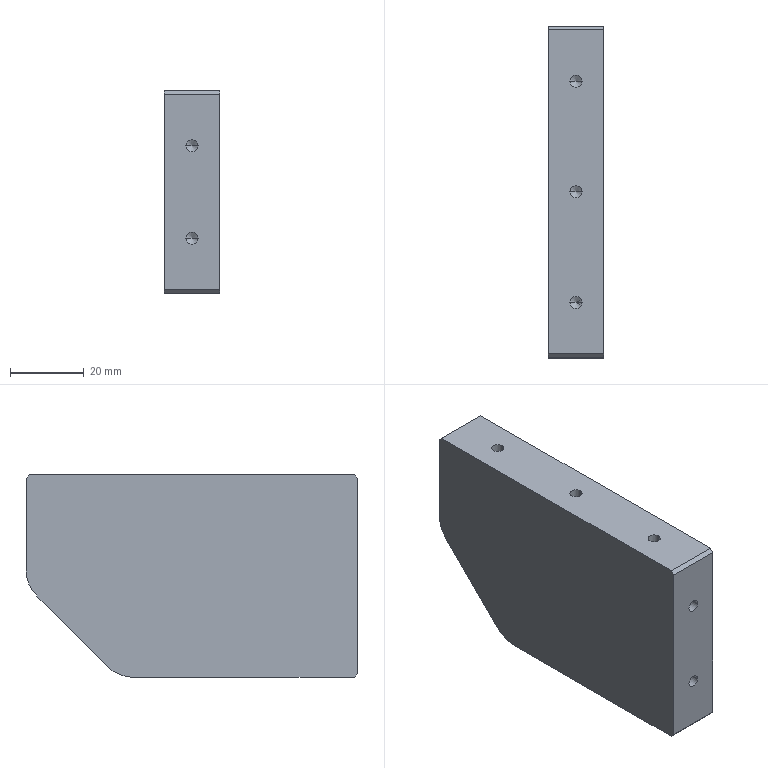Component | SolidWorks | 170423A4-PulleyPlateSupportBlock1-1 | 1 solid | 32 faces | box 15 x 90 x 55 mm | volume 68970 mm3 | cylinder 12 | cone 10 | plane 10 | commonest cylinder face diameters 3.3 x10 20 x2
build123d program:
from build123d import *

# Parameters (mm, degrees)
SKETCH1_W             = 55
SKETCH1_H             = 90
BOSS_EXTRUDE1_DEPTH   = 15
CHAMFER1_SIZE         = 25
FILLET1_R             = 10
M4_TAPPED_HOLE1_D     = 3.3
M4_TAPPED_HOLE1_DEPTH = 11.5
M4_TAPPED_HOLE1_TIP   = 0.9914
M4_TAPPED_HOLE2_D     = 3.3
M4_TAPPED_HOLE2_DEPTH = 11.5
M4_TAPPED_HOLE2_TIP   = 0.9914
CHAMFER2_SIZE         = 1


with BuildPart() as part:
    # Sketch1 → Boss-Extrude1 (new body)
    with BuildSketch(Plane.XY):
        with Locations((27.5, 45)):
            Rectangle(SKETCH1_W, SKETCH1_H)
    extrude(amount=BOSS_EXTRUDE1_DEPTH)

    # Chamfer1
    chamfer1_edges = [part.edges().sort_by_distance(p)[0] for p in [
        (55, 90, 7.5),
    ]]
    chamfer(chamfer1_edges, length=CHAMFER1_SIZE)

    # Fillet1
    fillet1_edges = [part.edges().sort_by_distance(p)[0] for p in [
        (30, 90, 7.5),
        (55, 65, 7.5),
    ]]
    fillet(fillet1_edges, radius=FILLET1_R)

    # M4 Tapped Hole1
    with Locations(Plane(origin=(0, 0, 0), x_dir=(-1, 0, 0), z_dir=(0, -1, 0))):
        with Locations((-40, -7.5), (-15, -7.5)):
            Hole(M4_TAPPED_HOLE1_D / 2, depth=M4_TAPPED_HOLE1_DEPTH)
            with Locations((0, 0, -(M4_TAPPED_HOLE1_DEPTH + M4_TAPPED_HOLE1_TIP / 2))):  # 118° drill point
                Cone(0, M4_TAPPED_HOLE1_D / 2, M4_TAPPED_HOLE1_TIP, mode=Mode.SUBTRACT)

    # M4 Tapped Hole2
    with Locations(Plane.ZY):
        with Locations((7.5, 15), (7.5, 75), (7.5, 45)):
            Hole(M4_TAPPED_HOLE2_D / 2, depth=M4_TAPPED_HOLE2_DEPTH)
            with Locations((0, 0, -(M4_TAPPED_HOLE2_DEPTH + M4_TAPPED_HOLE2_TIP / 2))):  # 118° drill point
                Cone(0, M4_TAPPED_HOLE2_D / 2, M4_TAPPED_HOLE2_TIP, mode=Mode.SUBTRACT)

    # Chamfer2
    chamfer2_edges = [part.edges().sort_by_distance(p)[0] for p in [
        (0, 90, 7.5),
        (55, 0, 7.5),
        (0, 0, 7.5),
    ]]
    chamfer(chamfer2_edges, length=CHAMFER2_SIZE)


solid = part.part

# Placed as in the assembly
solid = solid.moved(Location((139.754, -163.288, 409), (0, 90, 0)))
STEP:
#1=COLOUR_RGB('',0.7922,0.8196,0.9333);
#2=FILL_AREA_STYLE_COLOUR('',#1);
#3=FILL_AREA_STYLE('',(#2));
#4=SURFACE_STYLE_FILL_AREA(#3);
#5=SURFACE_SIDE_STYLE('',(#4));
#6=SURFACE_STYLE_USAGE(.BOTH.,#5);
#7=PRESENTATION_STYLE_ASSIGNMENT((#6));
#8=CARTESIAN_POINT('',(5.732,-3.476,15.65));
#9=VERTEX_POINT('',#8);
#10=CARTESIAN_POINT('',(5.862,-3.476,15.65));
#11=VERTEX_POINT('',#10);
#12=CARTESIAN_POINT('',(5.797,-3.476,15.65));
#13=DIRECTION('',(0.,0.,1.));
#14=DIRECTION('',(1.,0.,0.));
#15=AXIS2_PLACEMENT_3D('',#12,#13,#14);
#16=CIRCLE('',#15,0.06496);
#17=EDGE_CURVE('',#9,#11,#16,.T.);
#18=ORIENTED_EDGE('',*,*,#17,.F.);
#19=CARTESIAN_POINT('',(5.732,-3.476,16.102));
#20=VERTEX_POINT('',#19);
#21=CARTESIAN_POINT('',(5.732,-3.476,16.102));
#22=DIRECTION('',(0.,0.,1.));
#23=VECTOR('',#22,39.37);
#24=LINE('',#21,#23);
#25=EDGE_CURVE('',#9,#20,#24,.T.);
#26=ORIENTED_EDGE('',*,*,#25,.T.);
#27=CARTESIAN_POINT('',(5.862,-3.476,16.102));
#28=VERTEX_POINT('',#27);
#29=CARTESIAN_POINT('',(5.797,-3.476,16.102));
#30=DIRECTION('',(0.,0.,1.));
#31=DIRECTION('',(1.,0.,0.));
#32=AXIS2_PLACEMENT_3D('',#29,#30,#31);
#33=CIRCLE('',#32,0.06496);
#34=EDGE_CURVE('',#20,#28,#33,.T.);
#35=ORIENTED_EDGE('',*,*,#34,.T.);
#36=CARTESIAN_POINT('',(5.862,-3.476,16.102));
#37=DIRECTION('',(0.,0.,1.));
#38=VECTOR('',#37,39.37);
#39=LINE('',#36,#38);
#40=EDGE_CURVE('',#11,#28,#39,.T.);
#41=ORIENTED_EDGE('',*,*,#40,.F.);
#42=EDGE_LOOP('',(#18,#26,#35,#41));
#43=FACE_OUTER_BOUND('',#42,.T.);
#44=CARTESIAN_POINT('',(5.797,-3.476,16.102));
#45=DIRECTION('',(0.,0.,1.));
#46=DIRECTION('',(1.,0.,0.));
#47=AXIS2_PLACEMENT_3D('',#44,#45,#46);
#48=CYLINDRICAL_SURFACE('',#47,0.06496);
#49=ADVANCED_FACE('',(#43),#48,.F.);
#50=CARTESIAN_POINT('',(5.797,-3.476,15.611));
#51=VERTEX_POINT('',#50);
#52=CARTESIAN_POINT('',(5.862,-3.476,15.65));
#53=DIRECTION('',(0.8572,0.,0.515));
#54=VECTOR('',#53,39.37);
#55=LINE('',#52,#54);
#56=EDGE_CURVE('',#51,#11,#55,.T.);
#57=ORIENTED_EDGE('',*,*,#56,.F.);
#58=CARTESIAN_POINT('',(5.732,-3.476,15.65));
#59=DIRECTION('',(-0.8572,0.,0.515));
#60=VECTOR('',#59,39.37);
#61=LINE('',#58,#60);
#62=EDGE_CURVE('',#51,#9,#61,.T.);
#63=ORIENTED_EDGE('',*,*,#62,.T.);
#64=ORIENTED_EDGE('',*,*,#17,.T.);
#65=EDGE_LOOP('',(#57,#63,#64));
#66=FACE_OUTER_BOUND('',#65,.T.);
#67=CARTESIAN_POINT('',(5.797,-3.476,15.65));
#68=DIRECTION('',(0.,0.,1.));
#69=DIRECTION('',(1.,0.,0.));
#70=AXIS2_PLACEMENT_3D('',#67,#68,#69);
#71=CONICAL_SURFACE('',#70,0.06496,1.03);
#72=ADVANCED_FACE('',(#66),#71,.F.);
#73=CARTESIAN_POINT('',(5.732,-4.657,15.65));
#74=VERTEX_POINT('',#73);
#75=CARTESIAN_POINT('',(5.862,-4.657,15.65));
#76=VERTEX_POINT('',#75);
#77=CARTESIAN_POINT('',(5.797,-4.657,15.65));
#78=DIRECTION('',(0.,0.,1.));
#79=DIRECTION('',(1.,0.,0.));
#80=AXIS2_PLACEMENT_3D('',#77,#78,#79);
#81=CIRCLE('',#80,0.06496);
#82=EDGE_CURVE('',#74,#76,#81,.T.);
#83=ORIENTED_EDGE('',*,*,#82,.F.);
#84=CARTESIAN_POINT('',(5.732,-4.657,16.102));
#85=VERTEX_POINT('',#84);
#86=CARTESIAN_POINT('',(5.732,-4.657,16.102));
#87=DIRECTION('',(0.,0.,1.));
#88=VECTOR('',#87,39.37);
#89=LINE('',#86,#88);
#90=EDGE_CURVE('',#74,#85,#89,.T.);
#91=ORIENTED_EDGE('',*,*,#90,.T.);
#92=CARTESIAN_POINT('',(5.862,-4.657,16.102));
#93=VERTEX_POINT('',#92);
#94=CARTESIAN_POINT('',(5.797,-4.657,16.102));
#95=DIRECTION('',(0.,0.,1.));
#96=DIRECTION('',(1.,0.,0.));
#97=AXIS2_PLACEMENT_3D('',#94,#95,#96);
#98=CIRCLE('',#97,0.06496);
#99=EDGE_CURVE('',#85,#93,#98,.T.);
#100=ORIENTED_EDGE('',*,*,#99,.T.);
#101=CARTESIAN_POINT('',(5.862,-4.657,16.102));
#102=DIRECTION('',(0.,0.,1.));
#103=VECTOR('',#102,39.37);
#104=LINE('',#101,#103);
#105=EDGE_CURVE('',#76,#93,#104,.T.);
#106=ORIENTED_EDGE('',*,*,#105,.F.);
#107=EDGE_LOOP('',(#83,#91,#100,#106));
#108=FACE_OUTER_BOUND('',#107,.T.);
#109=CARTESIAN_POINT('',(5.797,-4.657,16.102));
#110=DIRECTION('',(0.,0.,1.));
#111=DIRECTION('',(1.,0.,0.));
#112=AXIS2_PLACEMENT_3D('',#109,#110,#111);
#113=CYLINDRICAL_SURFACE('',#112,0.06496);
#114=ADVANCED_FACE('',(#108),#113,.F.);
#115=CARTESIAN_POINT('',(5.797,-4.657,15.611));
#116=VERTEX_POINT('',#115);
#117=CARTESIAN_POINT('',(5.862,-4.657,15.65));
#118=DIRECTION('',(0.8572,0.,0.515));
#119=VECTOR('',#118,39.37);
#120=LINE('',#117,#119);
#121=EDGE_CURVE('',#116,#76,#120,.T.);
#122=ORIENTED_EDGE('',*,*,#121,.F.);
#123=CARTESIAN_POINT('',(5.732,-4.657,15.65));
#124=DIRECTION('',(-0.8572,0.,0.515));
#125=VECTOR('',#124,39.37);
#126=LINE('',#123,#125);
#127=EDGE_CURVE('',#116,#74,#126,.T.);
#128=ORIENTED_EDGE('',*,*,#127,.T.);
#129=ORIENTED_EDGE('',*,*,#82,.T.);
#130=EDGE_LOOP('',(#122,#128,#129));
#131=FACE_OUTER_BOUND('',#130,.T.);
#132=CARTESIAN_POINT('',(5.797,-4.657,15.65));
#133=DIRECTION('',(0.,0.,1.));
#134=DIRECTION('',(1.,0.,0.));
#135=AXIS2_PLACEMENT_3D('',#132,#133,#134);
#136=CONICAL_SURFACE('',#135,0.06496,1.03);
#137=ADVANCED_FACE('',(#131),#136,.F.);
#138=CARTESIAN_POINT('',(5.732,-5.838,15.65));
#139=VERTEX_POINT('',#138);
#140=CARTESIAN_POINT('',(5.862,-5.838,15.65));
#141=VERTEX_POINT('',#140);
#142=CARTESIAN_POINT('',(5.797,-5.838,15.65));
#143=DIRECTION('',(0.,0.,1.));
#144=DIRECTION('',(1.,0.,0.));
#145=AXIS2_PLACEMENT_3D('',#142,#143,#144);
#146=CIRCLE('',#145,0.06496);
#147=EDGE_CURVE('',#139,#141,#146,.T.);
#148=ORIENTED_EDGE('',*,*,#147,.F.);
#149=CARTESIAN_POINT('',(5.732,-5.838,16.102));
#150=VERTEX_POINT('',#149);
#151=CARTESIAN_POINT('',(5.732,-5.838,16.102));
#152=DIRECTION('',(0.,0.,1.));
#153=VECTOR('',#152,39.37);
#154=LINE('',#151,#153);
#155=EDGE_CURVE('',#139,#150,#154,.T.);
#156=ORIENTED_EDGE('',*,*,#155,.T.);
#157=CARTESIAN_POINT('',(5.862,-5.838,16.102));
#158=VERTEX_POINT('',#157);
#159=CARTESIAN_POINT('',(5.797,-5.838,16.102));
#160=DIRECTION('',(0.,0.,1.));
#161=DIRECTION('',(1.,0.,0.));
#162=AXIS2_PLACEMENT_3D('',#159,#160,#161);
#163=CIRCLE('',#162,0.06496);
#164=EDGE_CURVE('',#150,#158,#163,.T.);
#165=ORIENTED_EDGE('',*,*,#164,.T.);
#166=CARTESIAN_POINT('',(5.862,-5.838,16.102));
#167=DIRECTION('',(0.,0.,1.));
#168=VECTOR('',#167,39.37);
#169=LINE('',#166,#168);
#170=EDGE_CURVE('',#141,#158,#169,.T.);
#171=ORIENTED_EDGE('',*,*,#170,.F.);
#172=EDGE_LOOP('',(#148,#156,#165,#171));
#173=FACE_OUTER_BOUND('',#172,.T.);
#174=CARTESIAN_POINT('',(5.797,-5.838,16.102));
#175=DIRECTION('',(0.,0.,1.));
#176=DIRECTION('',(1.,0.,0.));
#177=AXIS2_PLACEMENT_3D('',#174,#175,#176);
#178=CYLINDRICAL_SURFACE('',#177,0.06496);
#179=ADVANCED_FACE('',(#173),#178,.F.);
#180=CARTESIAN_POINT('',(5.797,-5.838,15.611));
#181=VERTEX_POINT('',#180);
#182=CARTESIAN_POINT('',(5.862,-5.838,15.65));
#183=DIRECTION('',(0.8572,0.,0.515));
#184=VECTOR('',#183,39.37);
#185=LINE('',#182,#184);
#186=EDGE_CURVE('',#181,#141,#185,.T.);
#187=ORIENTED_EDGE('',*,*,#186,.F.);
#188=CARTESIAN_POINT('',(5.732,-5.838,15.65));
#189=DIRECTION('',(-0.8572,0.,0.515));
#190=VECTOR('',#189,39.37);
#191=LINE('',#188,#190);
#192=EDGE_CURVE('',#181,#139,#191,.T.);
#193=ORIENTED_EDGE('',*,*,#192,.T.);
#194=ORIENTED_EDGE('',*,*,#147,.T.);
#195=EDGE_LOOP('',(#187,#193,#194));
#196=FACE_OUTER_BOUND('',#195,.T.);
#197=CARTESIAN_POINT('',(5.797,-5.838,15.65));
#198=DIRECTION('',(0.,0.,1.));
#199=DIRECTION('',(1.,0.,0.));
#200=AXIS2_PLACEMENT_3D('',#197,#198,#199);
#201=CONICAL_SURFACE('',#200,0.06496,1.03);
#202=ADVANCED_FACE('',(#196),#201,.F.);
#203=CARTESIAN_POINT('',(5.862,-5.976,15.512));
#204=VERTEX_POINT('',#203);
#205=CARTESIAN_POINT('',(5.732,-5.976,15.512));
#206=VERTEX_POINT('',#205);
#207=CARTESIAN_POINT('',(5.797,-5.976,15.512));
#208=DIRECTION('',(0.,-1.,0.));
#209=DIRECTION('',(-1.,0.,0.));
#210=AXIS2_PLACEMENT_3D('',#207,#208,#209);
#211=CIRCLE('',#210,0.06496);
#212=EDGE_CURVE('',#204,#206,#211,.T.);
#213=ORIENTED_EDGE('',*,*,#212,.F.);
#214=CARTESIAN_POINT('',(5.862,-6.429,15.512));
#215=VERTEX_POINT('',#214);
#216=CARTESIAN_POINT('',(5.862,-6.429,15.512));
#217=DIRECTION('',(0.,-1.,0.));
#218=VECTOR('',#217,39.37);
#219=LINE('',#216,#218);
#220=EDGE_CURVE('',#204,#215,#219,.T.);
#221=ORIENTED_EDGE('',*,*,#220,.T.);
#222=CARTESIAN_POINT('',(5.732,-6.429,15.512));
#223=VERTEX_POINT('',#222);
#224=CARTESIAN_POINT('',(5.797,-6.429,15.512));
#225=DIRECTION('',(0.,-1.,0.));
#226=DIRECTION('',(-1.,0.,0.));
#227=AXIS2_PLACEMENT_3D('',#224,#225,#226);
#228=CIRCLE('',#227,0.06496);
#229=EDGE_CURVE('',#215,#223,#228,.T.);
#230=ORIENTED_EDGE('',*,*,#229,.T.);
#231=CARTESIAN_POINT('',(5.732,-6.429,15.512));
#232=DIRECTION('',(0.,-1.,0.));
#233=VECTOR('',#232,39.37);
#234=LINE('',#231,#233);
#235=EDGE_CURVE('',#206,#223,#234,.T.);
#236=ORIENTED_EDGE('',*,*,#235,.F.);
#237=EDGE_LOOP('',(#213,#221,#230,#236));
#238=FACE_OUTER_BOUND('',#237,.T.);
#239=CARTESIAN_POINT('',(5.797,-6.429,15.512));
#240=DIRECTION('',(0.,-1.,0.));
#241=DIRECTION('',(-1.,0.,0.));
#242=AXIS2_PLACEMENT_3D('',#239,#240,#241);
#243=CYLINDRICAL_SURFACE('',#242,0.06496);
#244=ADVANCED_FACE('',(#238),#243,.F.);
#245=CARTESIAN_POINT('',(5.797,-5.937,15.512));
#246=VERTEX_POINT('',#245);
#247=CARTESIAN_POINT('',(5.732,-5.976,15.512));
#248=DIRECTION('',(-0.8572,-0.515,0.));
#249=VECTOR('',#248,39.37);
#250=LINE('',#247,#249);
#251=EDGE_CURVE('',#246,#206,#250,.T.);
#252=ORIENTED_EDGE('',*,*,#251,.F.);
#253=CARTESIAN_POINT('',(5.862,-5.976,15.512));
#254=DIRECTION('',(0.8572,-0.515,-0.));
#255=VECTOR('',#254,39.37);
#256=LINE('',#253,#255);
#257=EDGE_CURVE('',#246,#204,#256,.T.);
#258=ORIENTED_EDGE('',*,*,#257,.T.);
#259=ORIENTED_EDGE('',*,*,#212,.T.);
#260=EDGE_LOOP('',(#252,#258,#259));
#261=FACE_OUTER_BOUND('',#260,.T.);
#262=CARTESIAN_POINT('',(5.797,-5.976,15.512));
#263=DIRECTION('',(0.,-1.,0.));
#264=DIRECTION('',(-1.,0.,0.));
#265=AXIS2_PLACEMENT_3D('',#262,#263,#264);
#266=CONICAL_SURFACE('',#265,0.06496,1.03);
#267=ADVANCED_FACE('',(#261),#266,.F.);
#268=CARTESIAN_POINT('',(5.862,-5.976,14.528));
#269=VERTEX_POINT('',#268);
#270=CARTESIAN_POINT('',(5.732,-5.976,14.528));
#271=VERTEX_POINT('',#270);
#272=CARTESIAN_POINT('',(5.797,-5.976,14.528));
#273=DIRECTION('',(0.,-1.,0.));
#274=DIRECTION('',(-1.,0.,0.));
#275=AXIS2_PLACEMENT_3D('',#272,#273,#274);
#276=CIRCLE('',#275,0.06496);
#277=EDGE_CURVE('',#269,#271,#276,.T.);
#278=ORIENTED_EDGE('',*,*,#277,.F.);
#279=CARTESIAN_POINT('',(5.862,-6.429,14.528));
#280=VERTEX_POINT('',#279);
#281=CARTESIAN_POINT('',(5.862,-6.429,14.528));
#282=DIRECTION('',(0.,-1.,0.));
#283=VECTOR('',#282,39.37);
#284=LINE('',#281,#283);
#285=EDGE_CURVE('',#269,#280,#284,.T.);
#286=ORIENTED_EDGE('',*,*,#285,.T.);
#287=CARTESIAN_POINT('',(5.732,-6.429,14.528));
#288=VERTEX_POINT('',#287);
#289=CARTESIAN_POINT('',(5.797,-6.429,14.528));
#290=DIRECTION('',(0.,-1.,0.));
#291=DIRECTION('',(-1.,0.,0.));
#292=AXIS2_PLACEMENT_3D('',#289,#290,#291);
#293=CIRCLE('',#292,0.06496);
#294=EDGE_CURVE('',#280,#288,#293,.T.);
#295=ORIENTED_EDGE('',*,*,#294,.T.);
#296=CARTESIAN_POINT('',(5.732,-6.429,14.528));
#297=DIRECTION('',(0.,-1.,0.));
#298=VECTOR('',#297,39.37);
#299=LINE('',#296,#298);
#300=EDGE_CURVE('',#271,#288,#299,.T.);
#301=ORIENTED_EDGE('',*,*,#300,.F.);
#302=EDGE_LOOP('',(#278,#286,#295,#301));
#303=FACE_OUTER_BOUND('',#302,.T.);
#304=CARTESIAN_POINT('',(5.797,-6.429,14.528));
#305=DIRECTION('',(0.,-1.,0.));
#306=DIRECTION('',(-1.,0.,0.));
#307=AXIS2_PLACEMENT_3D('',#304,#305,#306);
#308=CYLINDRICAL_SURFACE('',#307,0.06496);
#309=ADVANCED_FACE('',(#303),#308,.F.);
#310=CARTESIAN_POINT('',(5.797,-5.937,14.528));
#311=VERTEX_POINT('',#310);
#312=CARTESIAN_POINT('',(5.732,-5.976,14.528));
#313=DIRECTION('',(-0.8572,-0.515,0.));
#314=VECTOR('',#313,39.37);
#315=LINE('',#312,#314);
#316=EDGE_CURVE('',#311,#271,#315,.T.);
#317=ORIENTED_EDGE('',*,*,#316,.F.);
#318=CARTESIAN_POINT('',(5.862,-5.976,14.528));
#319=DIRECTION('',(0.8572,-0.515,-0.));
#320=VECTOR('',#319,39.37);
#321=LINE('',#318,#320);
#322=EDGE_CURVE('',#311,#269,#321,.T.);
#323=ORIENTED_EDGE('',*,*,#322,.T.);
#324=ORIENTED_EDGE('',*,*,#277,.T.);
#325=EDGE_LOOP('',(#317,#323,#324));
#326=FACE_OUTER_BOUND('',#325,.T.);
#327=CARTESIAN_POINT('',(5.797,-5.976,14.528));
#328=DIRECTION('',(0.,-1.,0.));
#329=DIRECTION('',(-1.,0.,0.));
#330=AXIS2_PLACEMENT_3D('',#327,#328,#329);
#331=CONICAL_SURFACE('',#330,0.06496,1.03);
#332=ADVANCED_FACE('',(#326),#331,.F.);
#333=CARTESIAN_POINT('',(5.797,-3.476,16.102));
#334=DIRECTION('',(0.,0.,1.));
#335=DIRECTION('',(1.,0.,0.));
#336=AXIS2_PLACEMENT_3D('',#333,#334,#335);
#337=CIRCLE('',#336,0.06496);
#338=EDGE_CURVE('',#28,#20,#337,.T.);
#339=ORIENTED_EDGE('',*,*,#338,.F.);
#340=ORIENTED_EDGE('',*,*,#34,.F.);
#341=EDGE_LOOP('',(#339,#340));
#342=FACE_BOUND('',#341,.T.);
#343=CARTESIAN_POINT('',(5.797,-4.657,16.102));
#344=DIRECTION('',(0.,0.,1.));
#345=DIRECTION('',(1.,0.,0.));
#346=AXIS2_PLACEMENT_3D('',#343,#344,#345);
#347=CIRCLE('',#346,0.06496);
#348=EDGE_CURVE('',#93,#85,#347,.T.);
#349=ORIENTED_EDGE('',*,*,#348,.F.);
#350=ORIENTED_EDGE('',*,*,#99,.F.);
#351=EDGE_LOOP('',(#349,#350));
#352=FACE_BOUND('',#351,.T.);
#353=CARTESIAN_POINT('',(5.797,-5.838,16.102));
#354=DIRECTION('',(0.,0.,1.));
#355=DIRECTION('',(1.,0.,0.));
#356=AXIS2_PLACEMENT_3D('',#353,#354,#355);
#357=CIRCLE('',#356,0.06496);
#358=EDGE_CURVE('',#158,#150,#357,.T.);
#359=ORIENTED_EDGE('',*,*,#358,.F.);
#360=ORIENTED_EDGE('',*,*,#164,.F.);
#361=EDGE_LOOP('',(#359,#360));
#362=FACE_BOUND('',#361,.T.);
#363=CARTESIAN_POINT('',(5.502,-2.925,16.102));
#364=VERTEX_POINT('',#363);
#365=CARTESIAN_POINT('',(5.502,-6.389,16.102));
#366=VERTEX_POINT('',#365);
#367=CARTESIAN_POINT('',(5.502,-6.429,16.102));
#368=DIRECTION('',(0.,-1.,0.));
#369=VECTOR('',#368,39.37);
#370=LINE('',#367,#369);
#371=EDGE_CURVE('',#364,#366,#370,.T.);
#372=ORIENTED_EDGE('',*,*,#371,.T.);
#373=CARTESIAN_POINT('',(6.093,-6.389,16.102));
#374=VERTEX_POINT('',#373);
#375=CARTESIAN_POINT('',(6.093,-6.389,16.102));
#376=DIRECTION('',(1.,0.,0.));
#377=VECTOR('',#376,39.37);
#378=LINE('',#375,#377);
#379=EDGE_CURVE('',#366,#374,#378,.T.);
#380=ORIENTED_EDGE('',*,*,#379,.T.);
#381=CARTESIAN_POINT('',(6.093,-2.925,16.102));
#382=VERTEX_POINT('',#381);
#383=CARTESIAN_POINT('',(6.093,-6.429,16.102));
#384=DIRECTION('',(0.,-1.,0.));
#385=VECTOR('',#384,39.37);
#386=LINE('',#383,#385);
#387=EDGE_CURVE('',#382,#374,#386,.T.);
#388=ORIENTED_EDGE('',*,*,#387,.F.);
#389=CARTESIAN_POINT('',(6.093,-2.925,16.102));
#390=DIRECTION('',(-1.,0.,0.));
#391=VECTOR('',#390,39.37);
#392=LINE('',#389,#391);
#393=EDGE_CURVE('',#382,#364,#392,.T.);
#394=ORIENTED_EDGE('',*,*,#393,.T.);
#395=EDGE_LOOP('',(#372,#380,#388,#394));
#396=FACE_OUTER_BOUND('',#395,.T.);
#397=CARTESIAN_POINT('',(6.093,-6.429,16.102));
#398=DIRECTION('',(0.,0.,-1.));
#399=DIRECTION('',(-1.,0.,0.));
#400=AXIS2_PLACEMENT_3D('',#397,#398,#399);
#401=PLANE('',#400);
#402=ADVANCED_FACE('',(#342,#352,#362,#396),#401,.F.);
#403=CARTESIAN_POINT('',(5.797,-6.429,15.512));
#404=DIRECTION('',(0.,-1.,0.));
#405=DIRECTION('',(-1.,0.,0.));
#406=AXIS2_PLACEMENT_3D('',#403,#404,#405);
#407=CIRCLE('',#406,0.06496);
#408=EDGE_CURVE('',#223,#215,#407,.T.);
#409=ORIENTED_EDGE('',*,*,#408,.F.);
#410=ORIENTED_EDGE('',*,*,#229,.F.);
#411=EDGE_LOOP('',(#409,#410));
#412=FACE_BOUND('',#411,.T.);
#413=CARTESIAN_POINT('',(5.797,-6.429,14.528));
#414=DIRECTION('',(0.,-1.,0.));
#415=DIRECTION('',(-1.,0.,0.));
#416=AXIS2_PLACEMENT_3D('',#413,#414,#415);
#417=CIRCLE('',#416,0.06496);
#418=EDGE_CURVE('',#288,#280,#417,.T.);
#419=ORIENTED_EDGE('',*,*,#418,.F.);
#420=ORIENTED_EDGE('',*,*,#294,.F.);
#421=EDGE_LOOP('',(#419,#420));
#422=FACE_BOUND('',#421,.T.);
#423=CARTESIAN_POINT('',(5.502,-6.429,16.063));
#424=VERTEX_POINT('',#423);
#425=CARTESIAN_POINT('',(5.502,-6.429,13.976));
#426=VERTEX_POINT('',#425);
#427=CARTESIAN_POINT('',(5.502,-6.429,16.102));
#428=DIRECTION('',(0.,0.,-1.));
#429=VECTOR('',#428,39.37);
#430=LINE('',#427,#429);
#431=EDGE_CURVE('',#424,#426,#430,.T.);
#432=ORIENTED_EDGE('',*,*,#431,.T.);
#433=CARTESIAN_POINT('',(6.093,-6.429,13.976));
#434=VERTEX_POINT('',#433);
#435=CARTESIAN_POINT('',(6.093,-6.429,13.976));
#436=DIRECTION('',(1.,0.,0.));
#437=VECTOR('',#436,39.37);
#438=LINE('',#435,#437);
#439=EDGE_CURVE('',#426,#434,#438,.T.);
#440=ORIENTED_EDGE('',*,*,#439,.T.);
#441=CARTESIAN_POINT('',(6.093,-6.429,16.063));
#442=VERTEX_POINT('',#441);
#443=CARTESIAN_POINT('',(6.093,-6.429,16.102));
#444=DIRECTION('',(0.,0.,-1.));
#445=VECTOR('',#444,39.37);
#446=LINE('',#443,#445);
#447=EDGE_CURVE('',#442,#434,#446,.T.);
#448=ORIENTED_EDGE('',*,*,#447,.F.);
#449=CARTESIAN_POINT('',(6.093,-6.429,16.063));
#450=DIRECTION('',(-1.,0.,0.));
#451=VECTOR('',#450,39.37);
#452=LINE('',#449,#451);
#453=EDGE_CURVE('',#442,#424,#452,.T.);
#454=ORIENTED_EDGE('',*,*,#453,.T.);
#455=EDGE_LOOP('',(#432,#440,#448,#454));
#456=FACE_OUTER_BOUND('',#455,.T.);
#457=CARTESIAN_POINT('',(6.093,-6.429,16.102));
#458=DIRECTION('',(0.,1.,0.));
#459=DIRECTION('',(1.,0.,0.));
#460=AXIS2_PLACEMENT_3D('',#457,#458,#459);
#461=PLANE('',#460);
#462=ADVANCED_FACE('',(#412,#422,#456),#461,.F.);
#463=CARTESIAN_POINT('',(6.093,-6.389,13.937));
#464=VERTEX_POINT('',#463);
#465=CARTESIAN_POINT('',(6.093,-4.033,13.937));
#466=VERTEX_POINT('',#465);
#467=CARTESIAN_POINT('',(6.093,-6.429,13.937));
#468=DIRECTION('',(0.,1.,0.));
#469=VECTOR('',#468,39.37);
#470=LINE('',#467,#469);
#471=EDGE_CURVE('',#464,#466,#470,.T.);
#472=ORIENTED_EDGE('',*,*,#471,.F.);
#473=CARTESIAN_POINT('',(5.502,-6.389,13.937));
#474=VERTEX_POINT('',#473);
#475=CARTESIAN_POINT('',(6.093,-6.389,13.937));
#476=DIRECTION('',(-1.,0.,0.));
#477=VECTOR('',#476,39.37);
#478=LINE('',#475,#477);
#479=EDGE_CURVE('',#464,#474,#478,.T.);
#480=ORIENTED_EDGE('',*,*,#479,.T.);
#481=CARTESIAN_POINT('',(5.502,-4.033,13.937));
#482=VERTEX_POINT('',#481);
#483=CARTESIAN_POINT('',(5.502,-6.429,13.937));
#484=DIRECTION('',(0.,1.,0.));
#485=VECTOR('',#484,39.37);
#486=LINE('',#483,#485);
#487=EDGE_CURVE('',#474,#482,#486,.T.);
#488=ORIENTED_EDGE('',*,*,#487,.T.);
#489=CARTESIAN_POINT('',(6.093,-4.033,13.937));
#490=DIRECTION('',(1.,0.,0.));
#491=VECTOR('',#490,39.37);
#492=LINE('',#489,#491);
#493=EDGE_CURVE('',#482,#466,#492,.T.);
#494=ORIENTED_EDGE('',*,*,#493,.T.);
#495=EDGE_LOOP('',(#472,#480,#488,#494));
#496=FACE_OUTER_BOUND('',#495,.T.);
#497=CARTESIAN_POINT('',(6.093,-6.429,13.937));
#498=DIRECTION('',(0.,0.,1.));
#499=DIRECTION('',(1.,0.,0.));
#500=AXIS2_PLACEMENT_3D('',#497,#498,#499);
#501=PLANE('',#500);
#502=ADVANCED_FACE('',(#496),#501,.F.);
#503=CARTESIAN_POINT('',(5.502,-2.885,15.084));
#504=VERTEX_POINT('',#503);
#505=CARTESIAN_POINT('',(5.502,-2.885,16.063));
#506=VERTEX_POINT('',#505);
#507=CARTESIAN_POINT('',(5.502,-2.885,16.102));
#508=DIRECTION('',(0.,0.,1.));
#509=VECTOR('',#508,39.37);
#510=LINE('',#507,#509);
#511=EDGE_CURVE('',#504,#506,#510,.T.);
#512=ORIENTED_EDGE('',*,*,#511,.T.);
#513=CARTESIAN_POINT('',(6.093,-2.885,16.063));
#514=VERTEX_POINT('',#513);
#515=CARTESIAN_POINT('',(6.093,-2.885,16.063));
#516=DIRECTION('',(1.,0.,0.));
#517=VECTOR('',#516,39.37);
#518=LINE('',#515,#517);
#519=EDGE_CURVE('',#506,#514,#518,.T.);
#520=ORIENTED_EDGE('',*,*,#519,.T.);
#521=CARTESIAN_POINT('',(6.093,-2.885,15.084));
#522=VERTEX_POINT('',#521);
#523=CARTESIAN_POINT('',(6.093,-2.885,16.102));
#524=DIRECTION('',(0.,0.,1.));
#525=VECTOR('',#524,39.37);
#526=LINE('',#523,#525);
#527=EDGE_CURVE('',#522,#514,#526,.T.);
#528=ORIENTED_EDGE('',*,*,#527,.F.);
#529=CARTESIAN_POINT('',(5.502,-2.885,15.084));
#530=DIRECTION('',(-1.,0.,0.));
#531=VECTOR('',#530,39.37);
#532=LINE('',#529,#531);
#533=EDGE_CURVE('',#522,#504,#532,.T.);
#534=ORIENTED_EDGE('',*,*,#533,.T.);
#535=EDGE_LOOP('',(#512,#520,#528,#534));
#536=FACE_OUTER_BOUND('',#535,.T.);
#537=CARTESIAN_POINT('',(6.093,-2.885,16.102));
#538=DIRECTION('',(0.,-1.,0.));
#539=DIRECTION('',(-1.,0.,0.));
#540=AXIS2_PLACEMENT_3D('',#537,#538,#539);
#541=PLANE('',#540);
#542=ADVANCED_FACE('',(#536),#541,.F.);
#543=ORIENTED_EDGE('',*,*,#447,.T.);
#544=CARTESIAN_POINT('',(6.093,-6.389,13.937));
#545=DIRECTION('',(0.,0.7071,-0.7071));
#546=VECTOR('',#545,39.37);
#547=LINE('',#544,#546);
#548=EDGE_CURVE('',#434,#464,#547,.T.);
#549=ORIENTED_EDGE('',*,*,#548,.T.);
#550=ORIENTED_EDGE('',*,*,#471,.T.);
#551=CARTESIAN_POINT('',(6.093,-3.754,14.052));
#552=VERTEX_POINT('',#551);
#553=CARTESIAN_POINT('',(6.093,-4.033,14.331));
#554=DIRECTION('',(1.,0.,0.));
#555=DIRECTION('',(0.,0.,1.));
#556=AXIS2_PLACEMENT_3D('',#553,#554,#555);
#557=CIRCLE('',#556,0.3937);
#558=EDGE_CURVE('',#466,#552,#557,.T.);
#559=ORIENTED_EDGE('',*,*,#558,.T.);
#560=CARTESIAN_POINT('',(6.093,-3.001,14.806));
#561=VERTEX_POINT('',#560);
#562=CARTESIAN_POINT('',(6.093,-2.885,14.921));
#563=DIRECTION('',(0.,0.7071,0.7071));
#564=VECTOR('',#563,39.37);
#565=LINE('',#562,#564);
#566=EDGE_CURVE('',#552,#561,#565,.T.);
#567=ORIENTED_EDGE('',*,*,#566,.T.);
#568=CARTESIAN_POINT('',(6.093,-3.279,15.084));
#569=DIRECTION('',(1.,0.,0.));
#570=DIRECTION('',(0.,0.,1.));
#571=AXIS2_PLACEMENT_3D('',#568,#569,#570);
#572=CIRCLE('',#571,0.3937);
#573=EDGE_CURVE('',#561,#522,#572,.T.);
#574=ORIENTED_EDGE('',*,*,#573,.T.);
#575=ORIENTED_EDGE('',*,*,#527,.T.);
#576=CARTESIAN_POINT('',(6.093,-2.925,16.102));
#577=DIRECTION('',(0.,-0.7071,0.7071));
#578=VECTOR('',#577,39.37);
#579=LINE('',#576,#578);
#580=EDGE_CURVE('',#514,#382,#579,.T.);
#581=ORIENTED_EDGE('',*,*,#580,.T.);
#582=ORIENTED_EDGE('',*,*,#387,.T.);
#583=CARTESIAN_POINT('',(6.093,-6.429,16.063));
#584=DIRECTION('',(0.,-0.7071,-0.7071));
#585=VECTOR('',#584,39.37);
#586=LINE('',#583,#585);
#587=EDGE_CURVE('',#374,#442,#586,.T.);
#588=ORIENTED_EDGE('',*,*,#587,.T.);
#589=EDGE_LOOP('',(#543,#549,#550,#559,#567,#574,#575,#581,#582,#588));
#590=FACE_OUTER_BOUND('',#589,.T.);
#591=CARTESIAN_POINT('',(6.093,-6.429,16.102));
#592=DIRECTION('',(-1.,0.,0.));
#593=DIRECTION('',(0.,0.,1.));
#594=AXIS2_PLACEMENT_3D('',#591,#592,#593);
#595=PLANE('',#594);
#596=ADVANCED_FACE('',(#590),#595,.F.);
#597=ORIENTED_EDGE('',*,*,#487,.F.);
#598=CARTESIAN_POINT('',(5.502,-7.492,15.039));
#599=DIRECTION('',(0.,-0.7071,0.7071));
#600=VECTOR('',#599,39.37);
#601=LINE('',#598,#600);
#602=EDGE_CURVE('',#474,#426,#601,.T.);
#603=ORIENTED_EDGE('',*,*,#602,.T.);
#604=ORIENTED_EDGE('',*,*,#431,.F.);
#605=CARTESIAN_POINT('',(5.502,-6.409,16.083));
#606=DIRECTION('',(0.,0.7071,0.7071));
#607=VECTOR('',#606,39.37);
#608=LINE('',#605,#607);
#609=EDGE_CURVE('',#424,#366,#608,.T.);
#610=ORIENTED_EDGE('',*,*,#609,.T.);
#611=ORIENTED_EDGE('',*,*,#371,.F.);
#612=CARTESIAN_POINT('',(5.502,-4.677,17.854));
#613=DIRECTION('',(0.,0.7071,-0.7071));
#614=VECTOR('',#613,39.37);
#615=LINE('',#612,#614);
#616=EDGE_CURVE('',#364,#506,#615,.T.);
#617=ORIENTED_EDGE('',*,*,#616,.T.);
#618=ORIENTED_EDGE('',*,*,#511,.F.);
#619=CARTESIAN_POINT('',(5.502,-3.001,14.806));
#620=VERTEX_POINT('',#619);
#621=CARTESIAN_POINT('',(5.502,-3.279,15.084));
#622=DIRECTION('',(-1.,0.,0.));
#623=DIRECTION('',(0.,0.,1.));
#624=AXIS2_PLACEMENT_3D('',#621,#622,#623);
#625=CIRCLE('',#624,0.3937);
#626=EDGE_CURVE('',#504,#620,#625,.T.);
#627=ORIENTED_EDGE('',*,*,#626,.T.);
#628=CARTESIAN_POINT('',(5.502,-3.754,14.052));
#629=VERTEX_POINT('',#628);
#630=CARTESIAN_POINT('',(5.502,-4.066,13.74));
#631=DIRECTION('',(0.,-0.7071,-0.7071));
#632=VECTOR('',#631,39.37);
#633=LINE('',#630,#632);
#634=EDGE_CURVE('',#620,#629,#633,.T.);
#635=ORIENTED_EDGE('',*,*,#634,.T.);
#636=CARTESIAN_POINT('',(5.502,-4.033,14.331));
#637=DIRECTION('',(-1.,0.,0.));
#638=DIRECTION('',(0.,0.,1.));
#639=AXIS2_PLACEMENT_3D('',#636,#637,#638);
#640=CIRCLE('',#639,0.3937);
#641=EDGE_CURVE('',#629,#482,#640,.T.);
#642=ORIENTED_EDGE('',*,*,#641,.T.);
#643=EDGE_LOOP('',(#597,#603,#604,#610,#611,#617,#618,#627,#635,#642));
#644=FACE_OUTER_BOUND('',#643,.T.);
#645=CARTESIAN_POINT('',(5.502,-6.429,16.102));
#646=DIRECTION('',(-1.,0.,0.));
#647=DIRECTION('',(0.,0.,1.));
#648=AXIS2_PLACEMENT_3D('',#645,#646,#647);
#649=PLANE('',#648);
#650=ADVANCED_FACE('',(#644),#649,.T.);
#651=ORIENTED_EDGE('',*,*,#566,.F.);
#652=CARTESIAN_POINT('',(5.502,-3.754,14.052));
#653=DIRECTION('',(-1.,0.,0.));
#654=VECTOR('',#653,39.37);
#655=LINE('',#652,#654);
#656=EDGE_CURVE('',#552,#629,#655,.T.);
#657=ORIENTED_EDGE('',*,*,#656,.T.);
#658=ORIENTED_EDGE('',*,*,#634,.F.);
#659=CARTESIAN_POINT('',(6.093,-3.001,14.806));
#660=DIRECTION('',(1.,0.,0.));
#661=VECTOR('',#660,39.37);
#662=LINE('',#659,#661);
#663=EDGE_CURVE('',#620,#561,#662,.T.);
#664=ORIENTED_EDGE('',*,*,#663,.T.);
#665=EDGE_LOOP('',(#651,#657,#658,#664));
#666=FACE_OUTER_BOUND('',#665,.T.);
#667=CARTESIAN_POINT('',(6.093,-2.885,14.921));
#668=DIRECTION('',(0.,-0.7071,0.7071));
#669=DIRECTION('',(-1.,0.,0.));
#670=AXIS2_PLACEMENT_3D('',#667,#668,#669);
#671=PLANE('',#670);
#672=ADVANCED_FACE('',(#666),#671,.F.);
#673=ORIENTED_EDGE('',*,*,#641,.F.);
#674=ORIENTED_EDGE('',*,*,#656,.F.);
#675=ORIENTED_EDGE('',*,*,#558,.F.);
#676=ORIENTED_EDGE('',*,*,#493,.F.);
#677=EDGE_LOOP('',(#673,#674,#675,#676));
#678=FACE_OUTER_BOUND('',#677,.T.);
#679=CARTESIAN_POINT('',(6.093,-4.033,14.331));
#680=DIRECTION('',(1.,0.,0.));
#681=DIRECTION('',(0.,0.,-1.));
#682=AXIS2_PLACEMENT_3D('',#679,#680,#681);
#683=CYLINDRICAL_SURFACE('',#682,0.3937);
#684=ADVANCED_FACE('',(#678),#683,.T.);
#685=ORIENTED_EDGE('',*,*,#573,.F.);
#686=ORIENTED_EDGE('',*,*,#663,.F.);
#687=ORIENTED_EDGE('',*,*,#626,.F.);
#688=ORIENTED_EDGE('',*,*,#533,.F.);
#689=EDGE_LOOP('',(#685,#686,#687,#688));
#690=FACE_OUTER_BOUND('',#689,.T.);
#691=CARTESIAN_POINT('',(6.093,-3.279,15.084));
#692=DIRECTION('',(-1.,0.,0.));
#693=DIRECTION('',(0.,0.,1.));
#694=AXIS2_PLACEMENT_3D('',#691,#692,#693);
#695=CYLINDRICAL_SURFACE('',#694,0.3937);
#696=ADVANCED_FACE('',(#690),#695,.T.);
#697=ORIENTED_EDGE('',*,*,#322,.F.);
#698=ORIENTED_EDGE('',*,*,#316,.T.);
#699=CARTESIAN_POINT('',(5.797,-5.976,14.528));
#700=DIRECTION('',(0.,-1.,0.));
#701=DIRECTION('',(-1.,0.,0.));
#702=AXIS2_PLACEMENT_3D('',#699,#700,#701);
#703=CIRCLE('',#702,0.06496);
#704=EDGE_CURVE('',#271,#269,#703,.T.);
#705=ORIENTED_EDGE('',*,*,#704,.T.);
#706=EDGE_LOOP('',(#697,#698,#705));
#707=FACE_OUTER_BOUND('',#706,.T.);
#708=CARTESIAN_POINT('',(5.797,-5.976,14.528));
#709=DIRECTION('',(0.,-1.,0.));
#710=DIRECTION('',(-1.,0.,0.));
#711=AXIS2_PLACEMENT_3D('',#708,#709,#710);
#712=CONICAL_SURFACE('',#711,0.06496,1.03);
#713=ADVANCED_FACE('',(#707),#712,.F.);
#714=ORIENTED_EDGE('',*,*,#285,.F.);
#715=ORIENTED_EDGE('',*,*,#704,.F.);
#716=ORIENTED_EDGE('',*,*,#300,.T.);
#717=ORIENTED_EDGE('',*,*,#418,.T.);
#718=EDGE_LOOP('',(#714,#715,#716,#717));
#719=FACE_OUTER_BOUND('',#718,.T.);
#720=CARTESIAN_POINT('',(5.797,-6.429,14.528));
#721=DIRECTION('',(0.,-1.,0.));
#722=DIRECTION('',(-1.,0.,0.));
#723=AXIS2_PLACEMENT_3D('',#720,#721,#722);
#724=CYLINDRICAL_SURFACE('',#723,0.06496);
#725=ADVANCED_FACE('',(#719),#724,.F.);
#726=ORIENTED_EDGE('',*,*,#257,.F.);
#727=ORIENTED_EDGE('',*,*,#251,.T.);
#728=CARTESIAN_POINT('',(5.797,-5.976,15.512));
#729=DIRECTION('',(0.,-1.,0.));
#730=DIRECTION('',(-1.,0.,0.));
#731=AXIS2_PLACEMENT_3D('',#728,#729,#730);
#732=CIRCLE('',#731,0.06496);
#733=EDGE_CURVE('',#206,#204,#732,.T.);
#734=ORIENTED_EDGE('',*,*,#733,.T.);
#735=EDGE_LOOP('',(#726,#727,#734));
#736=FACE_OUTER_BOUND('',#735,.T.);
#737=CARTESIAN_POINT('',(5.797,-5.976,15.512));
#738=DIRECTION('',(0.,-1.,0.));
#739=DIRECTION('',(-1.,0.,0.));
#740=AXIS2_PLACEMENT_3D('',#737,#738,#739);
#741=CONICAL_SURFACE('',#740,0.06496,1.03);
#742=ADVANCED_FACE('',(#736),#741,.F.);
#743=ORIENTED_EDGE('',*,*,#220,.F.);
#744=ORIENTED_EDGE('',*,*,#733,.F.);
#745=ORIENTED_EDGE('',*,*,#235,.T.);
#746=ORIENTED_EDGE('',*,*,#408,.T.);
#747=EDGE_LOOP('',(#743,#744,#745,#746));
#748=FACE_OUTER_BOUND('',#747,.T.);
#749=CARTESIAN_POINT('',(5.797,-6.429,15.512));
#750=DIRECTION('',(0.,-1.,0.));
#751=DIRECTION('',(-1.,0.,0.));
#752=AXIS2_PLACEMENT_3D('',#749,#750,#751);
#753=CYLINDRICAL_SURFACE('',#752,0.06496);
#754=ADVANCED_FACE('',(#748),#753,.F.);
#755=ORIENTED_EDGE('',*,*,#192,.F.);
#756=ORIENTED_EDGE('',*,*,#186,.T.);
#757=CARTESIAN_POINT('',(5.797,-5.838,15.65));
#758=DIRECTION('',(0.,0.,1.));
#759=DIRECTION('',(1.,0.,0.));
#760=AXIS2_PLACEMENT_3D('',#757,#758,#759);
#761=CIRCLE('',#760,0.06496);
#762=EDGE_CURVE('',#141,#139,#761,.T.);
#763=ORIENTED_EDGE('',*,*,#762,.T.);
#764=EDGE_LOOP('',(#755,#756,#763));
#765=FACE_OUTER_BOUND('',#764,.T.);
#766=CARTESIAN_POINT('',(5.797,-5.838,15.65));
#767=DIRECTION('',(0.,0.,1.));
#768=DIRECTION('',(1.,0.,0.));
#769=AXIS2_PLACEMENT_3D('',#766,#767,#768);
#770=CONICAL_SURFACE('',#769,0.06496,1.03);
#771=ADVANCED_FACE('',(#765),#770,.F.);
#772=ORIENTED_EDGE('',*,*,#155,.F.);
#773=ORIENTED_EDGE('',*,*,#762,.F.);
#774=ORIENTED_EDGE('',*,*,#170,.T.);
#775=ORIENTED_EDGE('',*,*,#358,.T.);
#776=EDGE_LOOP('',(#772,#773,#774,#775));
#777=FACE_OUTER_BOUND('',#776,.T.);
#778=CARTESIAN_POINT('',(5.797,-5.838,16.102));
#779=DIRECTION('',(0.,0.,1.));
#780=DIRECTION('',(1.,0.,0.));
#781=AXIS2_PLACEMENT_3D('',#778,#779,#780);
#782=CYLINDRICAL_SURFACE('',#781,0.06496);
#783=ADVANCED_FACE('',(#777),#782,.F.);
#784=ORIENTED_EDGE('',*,*,#127,.F.);
#785=ORIENTED_EDGE('',*,*,#121,.T.);
#786=CARTESIAN_POINT('',(5.797,-4.657,15.65));
#787=DIRECTION('',(0.,0.,1.));
#788=DIRECTION('',(1.,0.,0.));
#789=AXIS2_PLACEMENT_3D('',#786,#787,#788);
#790=CIRCLE('',#789,0.06496);
#791=EDGE_CURVE('',#76,#74,#790,.T.);
#792=ORIENTED_EDGE('',*,*,#791,.T.);
#793=EDGE_LOOP('',(#784,#785,#792));
#794=FACE_OUTER_BOUND('',#793,.T.);
#795=CARTESIAN_POINT('',(5.797,-4.657,15.65));
#796=DIRECTION('',(0.,0.,1.));
#797=DIRECTION('',(1.,0.,0.));
#798=AXIS2_PLACEMENT_3D('',#795,#796,#797);
#799=CONICAL_SURFACE('',#798,0.06496,1.03);
#800=ADVANCED_FACE('',(#794),#799,.F.);
#801=ORIENTED_EDGE('',*,*,#90,.F.);
#802=ORIENTED_EDGE('',*,*,#791,.F.);
#803=ORIENTED_EDGE('',*,*,#105,.T.);
#804=ORIENTED_EDGE('',*,*,#348,.T.);
#805=EDGE_LOOP('',(#801,#802,#803,#804));
#806=FACE_OUTER_BOUND('',#805,.T.);
#807=CARTESIAN_POINT('',(5.797,-4.657,16.102));
#808=DIRECTION('',(0.,0.,1.));
#809=DIRECTION('',(1.,0.,0.));
#810=AXIS2_PLACEMENT_3D('',#807,#808,#809);
#811=CYLINDRICAL_SURFACE('',#810,0.06496);
#812=ADVANCED_FACE('',(#806),#811,.F.);
#813=ORIENTED_EDGE('',*,*,#62,.F.);
#814=ORIENTED_EDGE('',*,*,#56,.T.);
#815=CARTESIAN_POINT('',(5.797,-3.476,15.65));
#816=DIRECTION('',(0.,0.,1.));
#817=DIRECTION('',(1.,0.,0.));
#818=AXIS2_PLACEMENT_3D('',#815,#816,#817);
#819=CIRCLE('',#818,0.06496);
#820=EDGE_CURVE('',#11,#9,#819,.T.);
#821=ORIENTED_EDGE('',*,*,#820,.T.);
#822=EDGE_LOOP('',(#813,#814,#821));
#823=FACE_OUTER_BOUND('',#822,.T.);
#824=CARTESIAN_POINT('',(5.797,-3.476,15.65));
#825=DIRECTION('',(0.,0.,1.));
#826=DIRECTION('',(1.,0.,0.));
#827=AXIS2_PLACEMENT_3D('',#824,#825,#826);
#828=CONICAL_SURFACE('',#827,0.06496,1.03);
#829=ADVANCED_FACE('',(#823),#828,.F.);
#830=ORIENTED_EDGE('',*,*,#25,.F.);
#831=ORIENTED_EDGE('',*,*,#820,.F.);
#832=ORIENTED_EDGE('',*,*,#40,.T.);
#833=ORIENTED_EDGE('',*,*,#338,.T.);
#834=EDGE_LOOP('',(#830,#831,#832,#833));
#835=FACE_OUTER_BOUND('',#834,.T.);
#836=CARTESIAN_POINT('',(5.797,-3.476,16.102));
#837=DIRECTION('',(0.,0.,1.));
#838=DIRECTION('',(1.,0.,0.));
#839=AXIS2_PLACEMENT_3D('',#836,#837,#838);
#840=CYLINDRICAL_SURFACE('',#839,0.06496);
#841=ADVANCED_FACE('',(#835),#840,.F.);
#842=ORIENTED_EDGE('',*,*,#548,.F.);
#843=ORIENTED_EDGE('',*,*,#439,.F.);
#844=ORIENTED_EDGE('',*,*,#602,.F.);
#845=ORIENTED_EDGE('',*,*,#479,.F.);
#846=EDGE_LOOP('',(#842,#843,#844,#845));
#847=FACE_OUTER_BOUND('',#846,.T.);
#848=CARTESIAN_POINT('',(6.093,-6.389,13.937));
#849=DIRECTION('',(0.,0.7071,0.7071));
#850=DIRECTION('',(-1.,0.,0.));
#851=AXIS2_PLACEMENT_3D('',#848,#849,#850);
#852=PLANE('',#851);
#853=ADVANCED_FACE('',(#847),#852,.F.);
#854=ORIENTED_EDGE('',*,*,#587,.F.);
#855=ORIENTED_EDGE('',*,*,#379,.F.);
#856=ORIENTED_EDGE('',*,*,#609,.F.);
#857=ORIENTED_EDGE('',*,*,#453,.F.);
#858=EDGE_LOOP('',(#854,#855,#856,#857));
#859=FACE_OUTER_BOUND('',#858,.T.);
#860=CARTESIAN_POINT('',(6.093,-6.429,16.063));
#861=DIRECTION('',(0.,0.7071,-0.7071));
#862=DIRECTION('',(-1.,0.,0.));
#863=AXIS2_PLACEMENT_3D('',#860,#861,#862);
#864=PLANE('',#863);
#865=ADVANCED_FACE('',(#859),#864,.F.);
#866=ORIENTED_EDGE('',*,*,#580,.F.);
#867=ORIENTED_EDGE('',*,*,#519,.F.);
#868=ORIENTED_EDGE('',*,*,#616,.F.);
#869=ORIENTED_EDGE('',*,*,#393,.F.);
#870=EDGE_LOOP('',(#866,#867,#868,#869));
#871=FACE_OUTER_BOUND('',#870,.T.);
#872=CARTESIAN_POINT('',(6.093,-2.925,16.102));
#873=DIRECTION('',(0.,-0.7071,-0.7071));
#874=DIRECTION('',(-1.,0.,0.));
#875=AXIS2_PLACEMENT_3D('',#872,#873,#874);
#876=PLANE('',#875);
#877=ADVANCED_FACE('',(#871),#876,.F.);
#878=CLOSED_SHELL('',(#49,#72,#114,#137,#179,#202,#244,#267,#309,#332,#402,#462,#502,#542,#596,#650,#672,#684,#696,#713,#725,#742,#754,#771,#783,#800,#812,#829,#841,#853,#865,#877));
#879=MANIFOLD_SOLID_BREP('',#878);
#880=STYLED_ITEM('',(#7),#879);
#881=PRESENTATION_LAYER_ASSIGNMENT('','',(#880));
#882=(LENGTH_UNIT()NAMED_UNIT(*)SI_UNIT($,.METRE.));
#883=LENGTH_MEASURE_WITH_UNIT(LENGTH_MEASURE(0.0254),#882);
#884=DIMENSIONAL_EXPONENTS(1.,0.,0.,0.,0.,0.,0.);
#885=(CONVERSION_BASED_UNIT('',#883)LENGTH_UNIT()NAMED_UNIT(#884));
#886=UNCERTAINTY_MEASURE_WITH_UNIT(LENGTH_MEASURE(0.00001),#885,'','');
#887=(NAMED_UNIT(*)PLANE_ANGLE_UNIT()SI_UNIT($,.RADIAN.));
#888=(NAMED_UNIT(*)SI_UNIT($,.STERADIAN.)SOLID_ANGLE_UNIT());
#889=(GEOMETRIC_REPRESENTATION_CONTEXT(3)GLOBAL_UNCERTAINTY_ASSIGNED_CONTEXT((#886))GLOBAL_UNIT_ASSIGNED_CONTEXT((#885,#887,#888))REPRESENTATION_CONTEXT('',''));
#890=MECHANICAL_DESIGN_GEOMETRIC_PRESENTATION_REPRESENTATION('',(#880),#889);
#891=CARTESIAN_POINT('',(0.,0.,0.));
#892=DIRECTION('',(0.,0.,1.));
#893=DIRECTION('',(1.,0.,0.));
#894=AXIS2_PLACEMENT_3D('',#891,#892,#893);
#895=(LENGTH_UNIT()NAMED_UNIT(*)SI_UNIT($,.METRE.));
#896=LENGTH_MEASURE_WITH_UNIT(LENGTH_MEASURE(0.0254),#895);
#897=DIMENSIONAL_EXPONENTS(1.,0.,0.,0.,0.,0.,0.);
#898=(CONVERSION_BASED_UNIT('',#896)LENGTH_UNIT()NAMED_UNIT(#897));
#899=UNCERTAINTY_MEASURE_WITH_UNIT(LENGTH_MEASURE(0.00001),#898,'','');
#900=(NAMED_UNIT(*)PLANE_ANGLE_UNIT()SI_UNIT($,.RADIAN.));
#901=(NAMED_UNIT(*)SI_UNIT($,.STERADIAN.)SOLID_ANGLE_UNIT());
#902=(GEOMETRIC_REPRESENTATION_CONTEXT(3)GLOBAL_UNCERTAINTY_ASSIGNED_CONTEXT((#899))GLOBAL_UNIT_ASSIGNED_CONTEXT((#898,#900,#901))REPRESENTATION_CONTEXT('',''));
#903=ADVANCED_BREP_SHAPE_REPRESENTATION('',(#879,#894),#902);